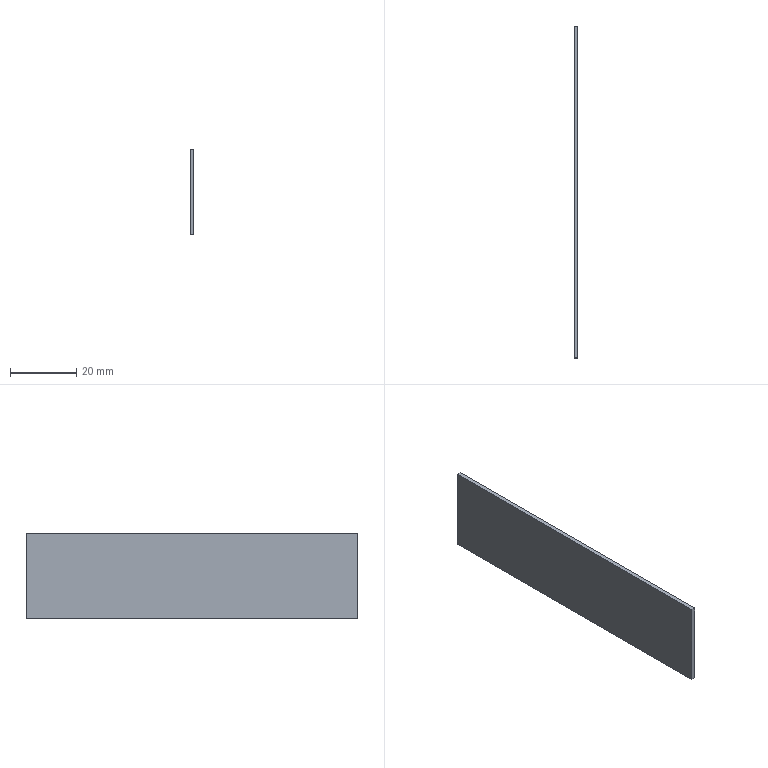Component | SolidWorks | 27x100IronPlate-2 | 1 solid | 6 faces | box 1.2 x 100 x 25.8 mm | volume 3096 mm3 | plane 6
STEP:
#1=COLOUR_RGB('',0.7922,0.8196,0.9333);
#2=FILL_AREA_STYLE_COLOUR('',#1);
#3=FILL_AREA_STYLE('',(#2));
#4=SURFACE_STYLE_FILL_AREA(#3);
#5=SURFACE_SIDE_STYLE('',(#4));
#6=SURFACE_STYLE_USAGE(.BOTH.,#5);
#7=PRESENTATION_STYLE_ASSIGNMENT((#6));
#8=CARTESIAN_POINT('',(19.685,62.992,9.024));
#9=VERTEX_POINT('',#8);
#10=CARTESIAN_POINT('',(19.685,66.929,9.024));
#11=VERTEX_POINT('',#10);
#12=CARTESIAN_POINT('',(19.685,66.929,9.024));
#13=DIRECTION('',(0.,1.,0.));
#14=VECTOR('',#13,39.37);
#15=LINE('',#12,#14);
#16=EDGE_CURVE('',#9,#11,#15,.T.);
#17=ORIENTED_EDGE('',*,*,#16,.F.);
#18=CARTESIAN_POINT('',(19.638,62.992,9.024));
#19=VERTEX_POINT('',#18);
#20=CARTESIAN_POINT('',(19.638,62.992,9.024));
#21=DIRECTION('',(1.,0.,0.));
#22=VECTOR('',#21,39.37);
#23=LINE('',#20,#22);
#24=EDGE_CURVE('',#19,#9,#23,.T.);
#25=ORIENTED_EDGE('',*,*,#24,.F.);
#26=CARTESIAN_POINT('',(19.638,66.929,9.024));
#27=VERTEX_POINT('',#26);
#28=CARTESIAN_POINT('',(19.638,66.929,9.024));
#29=DIRECTION('',(0.,1.,0.));
#30=VECTOR('',#29,39.37);
#31=LINE('',#28,#30);
#32=EDGE_CURVE('',#19,#27,#31,.T.);
#33=ORIENTED_EDGE('',*,*,#32,.T.);
#34=CARTESIAN_POINT('',(19.638,66.929,9.024));
#35=DIRECTION('',(1.,0.,0.));
#36=VECTOR('',#35,39.37);
#37=LINE('',#34,#36);
#38=EDGE_CURVE('',#27,#11,#37,.T.);
#39=ORIENTED_EDGE('',*,*,#38,.T.);
#40=EDGE_LOOP('',(#17,#25,#33,#39));
#41=FACE_OUTER_BOUND('',#40,.T.);
#42=CARTESIAN_POINT('',(19.638,66.929,9.024));
#43=DIRECTION('',(0.,0.,-1.));
#44=DIRECTION('',(0.,1.,0.));
#45=AXIS2_PLACEMENT_3D('',#42,#43,#44);
#46=PLANE('',#45);
#47=ADVANCED_FACE('',(#41),#46,.T.);
#48=CARTESIAN_POINT('',(19.685,62.992,10.039));
#49=VERTEX_POINT('',#48);
#50=CARTESIAN_POINT('',(19.685,62.992,10.039));
#51=DIRECTION('',(0.,0.,-1.));
#52=VECTOR('',#51,39.37);
#53=LINE('',#50,#52);
#54=EDGE_CURVE('',#49,#9,#53,.T.);
#55=ORIENTED_EDGE('',*,*,#54,.F.);
#56=CARTESIAN_POINT('',(19.638,62.992,10.039));
#57=VERTEX_POINT('',#56);
#58=CARTESIAN_POINT('',(19.638,62.992,10.039));
#59=DIRECTION('',(1.,0.,0.));
#60=VECTOR('',#59,39.37);
#61=LINE('',#58,#60);
#62=EDGE_CURVE('',#57,#49,#61,.T.);
#63=ORIENTED_EDGE('',*,*,#62,.F.);
#64=CARTESIAN_POINT('',(19.638,62.992,10.039));
#65=DIRECTION('',(0.,0.,-1.));
#66=VECTOR('',#65,39.37);
#67=LINE('',#64,#66);
#68=EDGE_CURVE('',#57,#19,#67,.T.);
#69=ORIENTED_EDGE('',*,*,#68,.T.);
#70=ORIENTED_EDGE('',*,*,#24,.T.);
#71=EDGE_LOOP('',(#55,#63,#69,#70));
#72=FACE_OUTER_BOUND('',#71,.T.);
#73=CARTESIAN_POINT('',(19.638,62.992,10.039));
#74=DIRECTION('',(0.,-1.,0.));
#75=DIRECTION('',(0.,0.,-1.));
#76=AXIS2_PLACEMENT_3D('',#73,#74,#75);
#77=PLANE('',#76);
#78=ADVANCED_FACE('',(#72),#77,.T.);
#79=CARTESIAN_POINT('',(19.685,66.929,10.039));
#80=VERTEX_POINT('',#79);
#81=CARTESIAN_POINT('',(19.685,66.929,10.039));
#82=DIRECTION('',(0.,-1.,-0.));
#83=VECTOR('',#82,39.37);
#84=LINE('',#81,#83);
#85=EDGE_CURVE('',#80,#49,#84,.T.);
#86=ORIENTED_EDGE('',*,*,#85,.F.);
#87=CARTESIAN_POINT('',(19.638,66.929,10.039));
#88=VERTEX_POINT('',#87);
#89=CARTESIAN_POINT('',(19.638,66.929,10.039));
#90=DIRECTION('',(1.,0.,0.));
#91=VECTOR('',#90,39.37);
#92=LINE('',#89,#91);
#93=EDGE_CURVE('',#88,#80,#92,.T.);
#94=ORIENTED_EDGE('',*,*,#93,.F.);
#95=CARTESIAN_POINT('',(19.638,66.929,10.039));
#96=DIRECTION('',(0.,-1.,-0.));
#97=VECTOR('',#96,39.37);
#98=LINE('',#95,#97);
#99=EDGE_CURVE('',#88,#57,#98,.T.);
#100=ORIENTED_EDGE('',*,*,#99,.T.);
#101=ORIENTED_EDGE('',*,*,#62,.T.);
#102=EDGE_LOOP('',(#86,#94,#100,#101));
#103=FACE_OUTER_BOUND('',#102,.T.);
#104=CARTESIAN_POINT('',(19.638,66.929,10.039));
#105=DIRECTION('',(0.,-0.,1.));
#106=DIRECTION('',(0.,-1.,-0.));
#107=AXIS2_PLACEMENT_3D('',#104,#105,#106);
#108=PLANE('',#107);
#109=ADVANCED_FACE('',(#103),#108,.T.);
#110=CARTESIAN_POINT('',(19.685,66.929,10.039));
#111=DIRECTION('',(0.,0.,1.));
#112=VECTOR('',#111,39.37);
#113=LINE('',#110,#112);
#114=EDGE_CURVE('',#11,#80,#113,.T.);
#115=ORIENTED_EDGE('',*,*,#114,.F.);
#116=ORIENTED_EDGE('',*,*,#38,.F.);
#117=CARTESIAN_POINT('',(19.638,66.929,10.039));
#118=DIRECTION('',(0.,0.,1.));
#119=VECTOR('',#118,39.37);
#120=LINE('',#117,#119);
#121=EDGE_CURVE('',#27,#88,#120,.T.);
#122=ORIENTED_EDGE('',*,*,#121,.T.);
#123=ORIENTED_EDGE('',*,*,#93,.T.);
#124=EDGE_LOOP('',(#115,#116,#122,#123));
#125=FACE_OUTER_BOUND('',#124,.T.);
#126=CARTESIAN_POINT('',(19.638,66.929,10.039));
#127=DIRECTION('',(0.,1.,0.));
#128=DIRECTION('',(0.,0.,1.));
#129=AXIS2_PLACEMENT_3D('',#126,#127,#128);
#130=PLANE('',#129);
#131=ADVANCED_FACE('',(#125),#130,.T.);
#132=ORIENTED_EDGE('',*,*,#32,.F.);
#133=ORIENTED_EDGE('',*,*,#68,.F.);
#134=ORIENTED_EDGE('',*,*,#99,.F.);
#135=ORIENTED_EDGE('',*,*,#121,.F.);
#136=EDGE_LOOP('',(#132,#133,#134,#135));
#137=FACE_OUTER_BOUND('',#136,.T.);
#138=CARTESIAN_POINT('',(19.638,64.961,9.531));
#139=DIRECTION('',(1.,0.,0.));
#140=DIRECTION('',(0.,0.,-1.));
#141=AXIS2_PLACEMENT_3D('',#138,#139,#140);
#142=PLANE('',#141);
#143=ADVANCED_FACE('',(#137),#142,.F.);
#144=ORIENTED_EDGE('',*,*,#16,.T.);
#145=ORIENTED_EDGE('',*,*,#114,.T.);
#146=ORIENTED_EDGE('',*,*,#85,.T.);
#147=ORIENTED_EDGE('',*,*,#54,.T.);
#148=EDGE_LOOP('',(#144,#145,#146,#147));
#149=FACE_OUTER_BOUND('',#148,.T.);
#150=CARTESIAN_POINT('',(19.685,64.961,9.531));
#151=DIRECTION('',(1.,0.,0.));
#152=DIRECTION('',(0.,0.,-1.));
#153=AXIS2_PLACEMENT_3D('',#150,#151,#152);
#154=PLANE('',#153);
#155=ADVANCED_FACE('',(#149),#154,.T.);
#156=CLOSED_SHELL('',(#47,#78,#109,#131,#143,#155));
#157=MANIFOLD_SOLID_BREP('',#156);
#158=STYLED_ITEM('',(#7),#157);
#159=PRESENTATION_LAYER_ASSIGNMENT('','',(#158));
#160=CARTESIAN_POINT('',(0.,0.,0.));
#161=DIRECTION('',(0.,0.,1.));
#162=DIRECTION('',(1.,0.,0.));
#163=AXIS2_PLACEMENT_3D('',#160,#161,#162);
#164=(LENGTH_UNIT()NAMED_UNIT(*)SI_UNIT($,.METRE.));
#165=LENGTH_MEASURE_WITH_UNIT(LENGTH_MEASURE(0.0254),#164);
#166=DIMENSIONAL_EXPONENTS(1.,0.,0.,0.,0.,0.,0.);
#167=(CONVERSION_BASED_UNIT('',#165)LENGTH_UNIT()NAMED_UNIT(#166));
#168=UNCERTAINTY_MEASURE_WITH_UNIT(LENGTH_MEASURE(0.00001),#167,'','');
#169=(NAMED_UNIT(*)PLANE_ANGLE_UNIT()SI_UNIT($,.RADIAN.));
#170=(NAMED_UNIT(*)SI_UNIT($,.STERADIAN.)SOLID_ANGLE_UNIT());
#171=(GEOMETRIC_REPRESENTATION_CONTEXT(3)GLOBAL_UNCERTAINTY_ASSIGNED_CONTEXT((#168))GLOBAL_UNIT_ASSIGNED_CONTEXT((#167,#169,#170))REPRESENTATION_CONTEXT('',''));
#172=ADVANCED_BREP_SHAPE_REPRESENTATION('',(#157,#163),#171);
#173=(LENGTH_UNIT()NAMED_UNIT(*)SI_UNIT($,.METRE.));
#174=LENGTH_MEASURE_WITH_UNIT(LENGTH_MEASURE(0.0254),#173);
#175=DIMENSIONAL_EXPONENTS(1.,0.,0.,0.,0.,0.,0.);
#176=(CONVERSION_BASED_UNIT('',#174)LENGTH_UNIT()NAMED_UNIT(#175));
#177=UNCERTAINTY_MEASURE_WITH_UNIT(LENGTH_MEASURE(0.00001),#176,'','');
#178=(NAMED_UNIT(*)PLANE_ANGLE_UNIT()SI_UNIT($,.RADIAN.));
#179=(NAMED_UNIT(*)SI_UNIT($,.STERADIAN.)SOLID_ANGLE_UNIT());
#180=(GEOMETRIC_REPRESENTATION_CONTEXT(3)GLOBAL_UNCERTAINTY_ASSIGNED_CONTEXT((#177))GLOBAL_UNIT_ASSIGNED_CONTEXT((#176,#178,#179))REPRESENTATION_CONTEXT('',''));
#181=MECHANICAL_DESIGN_GEOMETRIC_PRESENTATION_REPRESENTATION('',(#158),#180);